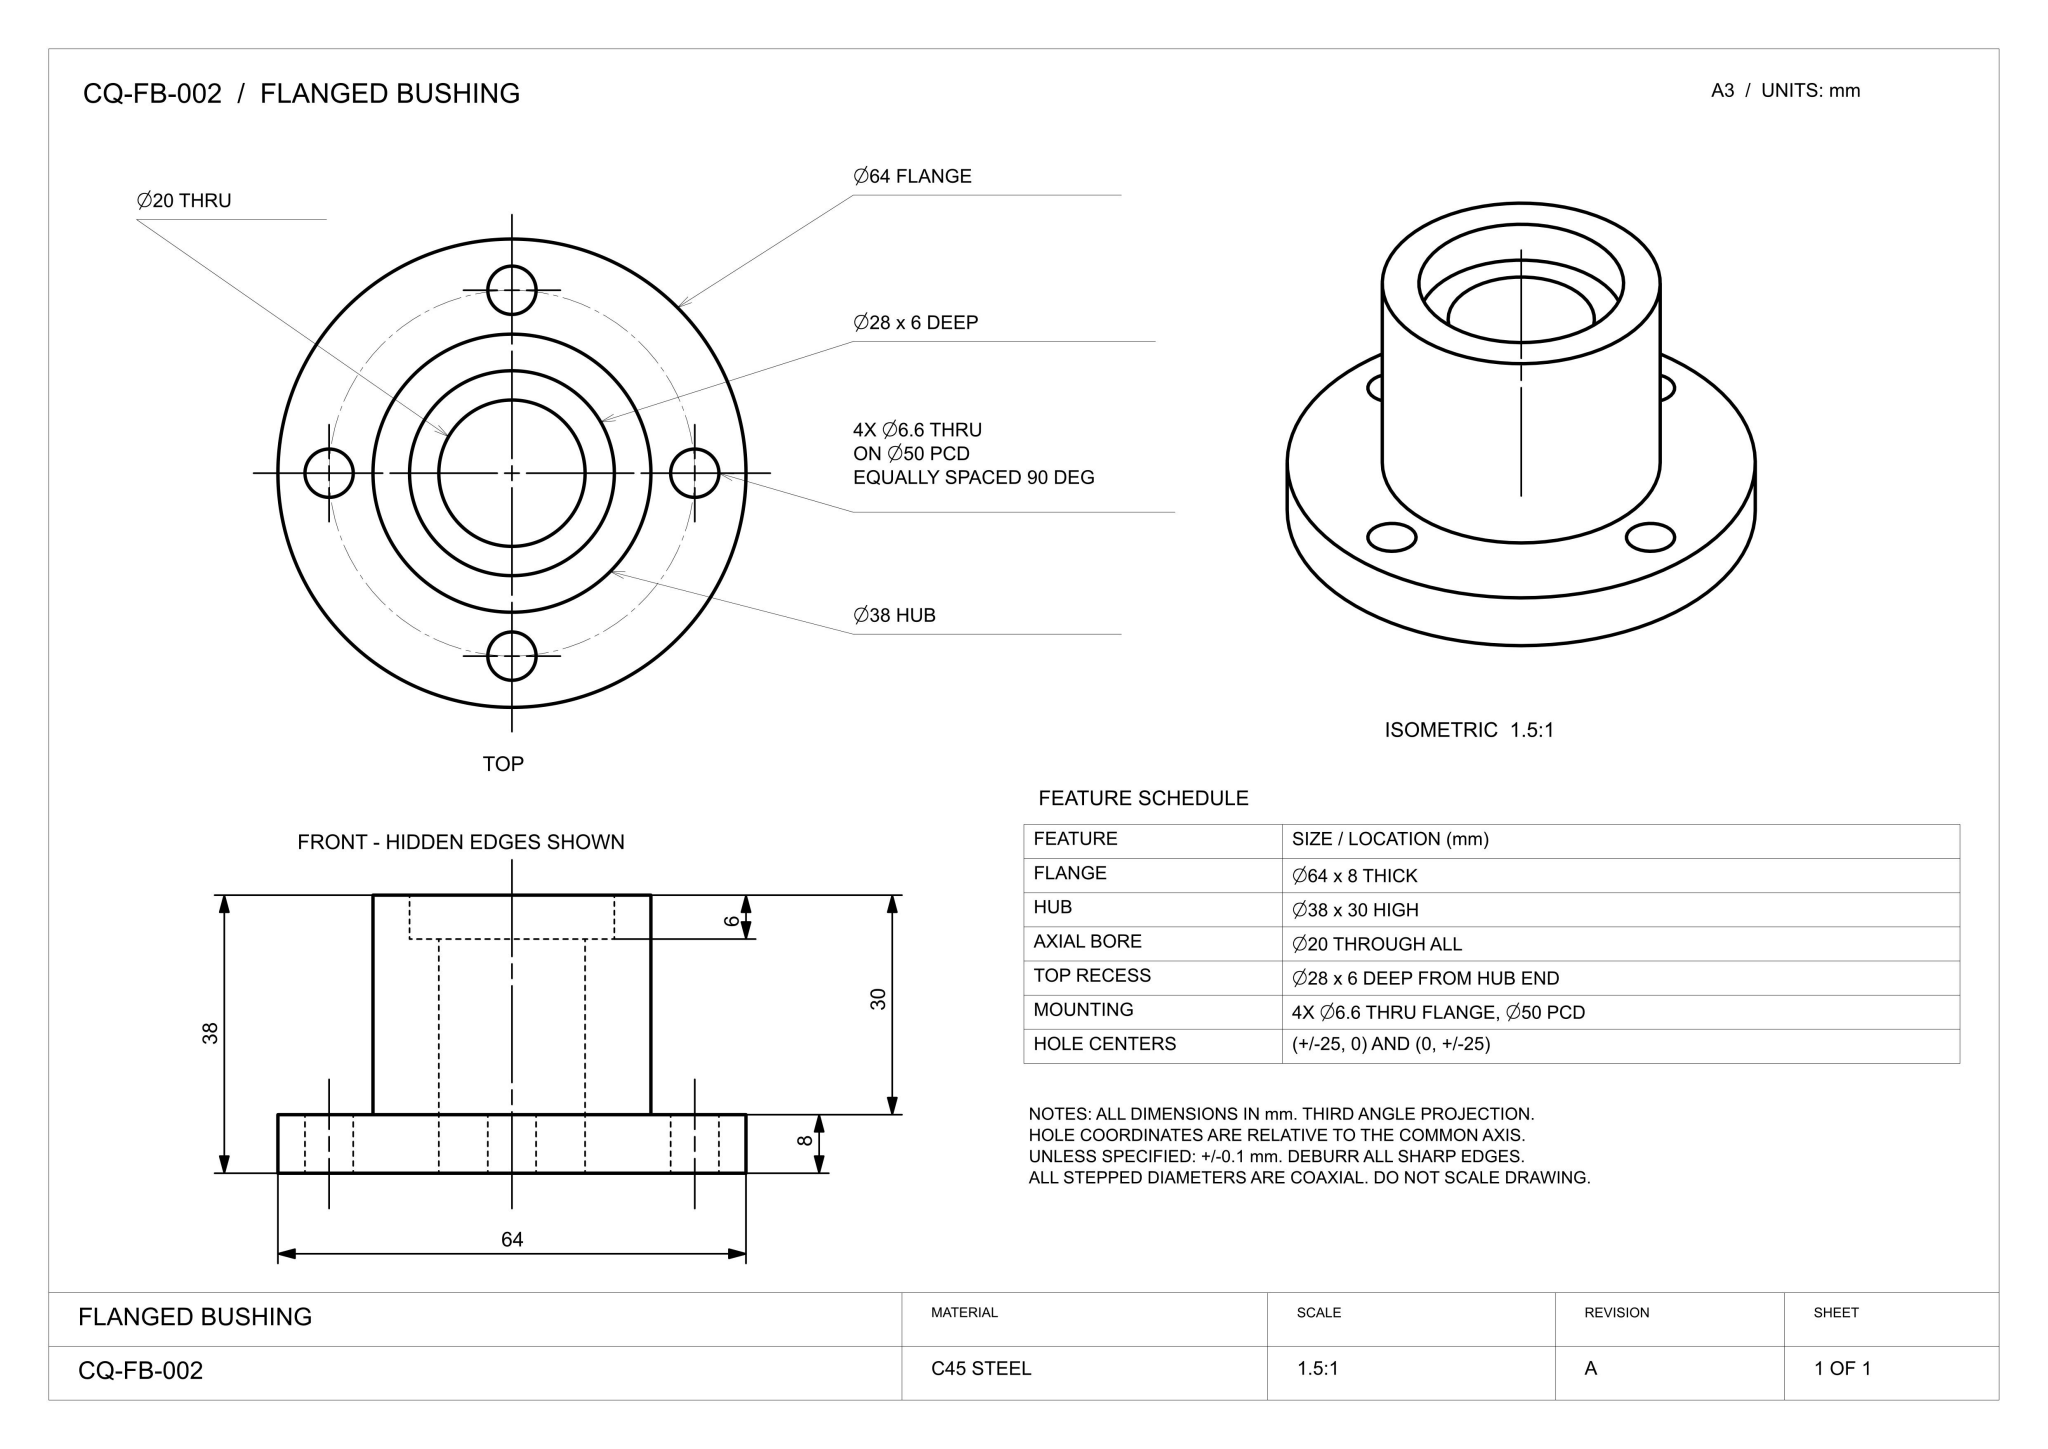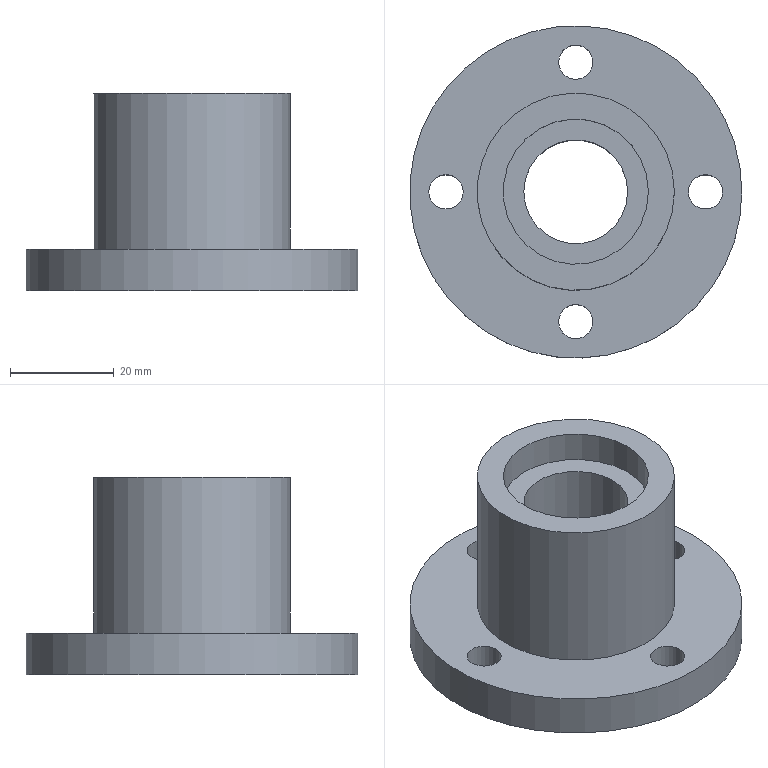Part | NX | mm | 1 solid | 12 faces | box 64 x 64 x 38 mm | volume 44917 mm3 | cylinder 8 | plane 4 | commonest cylinder face diameters 6.6 x4 64 x1 38 x1 20 x1 28 x1
STEP:
#1=CARTESIAN_POINT('',(0.,0.,0.));
#2=DIRECTION('',(0.,0.,1.));
#3=DIRECTION('',(1.,0.,0.));
#4=AXIS2_PLACEMENT_3D('',#1,#2,#3);
#5=(LENGTH_UNIT()NAMED_UNIT(*)SI_UNIT(.MILLI.,.METRE.));
#6=UNCERTAINTY_MEASURE_WITH_UNIT(LENGTH_MEASURE(0.00002),#5,'','');
#7=(NAMED_UNIT(*)PLANE_ANGLE_UNIT()SI_UNIT($,.RADIAN.));
#8=PLANE_ANGLE_MEASURE_WITH_UNIT(PLANE_ANGLE_MEASURE(0.01745),#7);
#9=DIMENSIONAL_EXPONENTS(0.,0.,0.,0.,0.,0.,0.);
#10=(CONVERSION_BASED_UNIT('',#8)NAMED_UNIT(#9)PLANE_ANGLE_UNIT());
#11=(NAMED_UNIT(*)SI_UNIT($,.STERADIAN.)SOLID_ANGLE_UNIT());
#12=(GEOMETRIC_REPRESENTATION_CONTEXT(3)GLOBAL_UNCERTAINTY_ASSIGNED_CONTEXT((#6))GLOBAL_UNIT_ASSIGNED_CONTEXT((#5,#10,#11))REPRESENTATION_CONTEXT('',''));
#13=SHAPE_REPRESENTATION('',(#4),#12);
#14=CARTESIAN_POINT('',(3.3,-25.,8.));
#15=VERTEX_POINT('',#14);
#16=CARTESIAN_POINT('',(0.,-25.,8.));
#17=DIRECTION('',(0.,0.,-1.));
#18=DIRECTION('',(1.,0.,0.));
#19=AXIS2_PLACEMENT_3D('',#16,#17,#18);
#20=CIRCLE('',#19,3.3);
#21=EDGE_CURVE('',#15,#15,#20,.T.);
#22=ORIENTED_EDGE('',*,*,#21,.T.);
#23=EDGE_LOOP('',(#22));
#24=FACE_BOUND('',#23,.T.);
#25=CARTESIAN_POINT('',(-21.7,0.,8.));
#26=VERTEX_POINT('',#25);
#27=CARTESIAN_POINT('',(-25.,0.,8.));
#28=DIRECTION('',(0.,0.,-1.));
#29=DIRECTION('',(1.,0.,0.));
#30=AXIS2_PLACEMENT_3D('',#27,#28,#29);
#31=CIRCLE('',#30,3.3);
#32=EDGE_CURVE('',#26,#26,#31,.T.);
#33=ORIENTED_EDGE('',*,*,#32,.T.);
#34=EDGE_LOOP('',(#33));
#35=FACE_BOUND('',#34,.T.);
#36=CARTESIAN_POINT('',(3.3,25.,8.));
#37=VERTEX_POINT('',#36);
#38=CARTESIAN_POINT('',(0.,25.,8.));
#39=DIRECTION('',(0.,0.,-1.));
#40=DIRECTION('',(1.,0.,0.));
#41=AXIS2_PLACEMENT_3D('',#38,#39,#40);
#42=CIRCLE('',#41,3.3);
#43=EDGE_CURVE('',#37,#37,#42,.T.);
#44=ORIENTED_EDGE('',*,*,#43,.T.);
#45=EDGE_LOOP('',(#44));
#46=FACE_BOUND('',#45,.T.);
#47=CARTESIAN_POINT('',(28.3,0.,8.));
#48=VERTEX_POINT('',#47);
#49=CARTESIAN_POINT('',(25.,0.,8.));
#50=DIRECTION('',(0.,0.,-1.));
#51=DIRECTION('',(1.,0.,0.));
#52=AXIS2_PLACEMENT_3D('',#49,#50,#51);
#53=CIRCLE('',#52,3.3);
#54=EDGE_CURVE('',#48,#48,#53,.T.);
#55=ORIENTED_EDGE('',*,*,#54,.T.);
#56=EDGE_LOOP('',(#55));
#57=FACE_BOUND('',#56,.T.);
#58=CARTESIAN_POINT('',(19.,0.,8.));
#59=VERTEX_POINT('',#58);
#60=CARTESIAN_POINT('',(0.,0.,8.));
#61=DIRECTION('',(0.,0.,1.));
#62=DIRECTION('',(1.,0.,0.));
#63=AXIS2_PLACEMENT_3D('',#60,#61,#62);
#64=CIRCLE('',#63,19.);
#65=EDGE_CURVE('',#59,#59,#64,.T.);
#66=ORIENTED_EDGE('',*,*,#65,.F.);
#67=EDGE_LOOP('',(#66));
#68=FACE_BOUND('',#67,.T.);
#69=CARTESIAN_POINT('',(32.,0.,8.));
#70=VERTEX_POINT('',#69);
#71=CARTESIAN_POINT('',(0.,0.,8.));
#72=DIRECTION('',(0.,0.,-1.));
#73=DIRECTION('',(1.,0.,0.));
#74=AXIS2_PLACEMENT_3D('',#71,#72,#73);
#75=CIRCLE('',#74,32.);
#76=EDGE_CURVE('',#70,#70,#75,.T.);
#77=ORIENTED_EDGE('',*,*,#76,.F.);
#78=EDGE_LOOP('',(#77));
#79=FACE_BOUND('',#78,.T.);
#80=CARTESIAN_POINT('',(0.,0.,8.));
#81=DIRECTION('',(0.,0.,1.));
#82=DIRECTION('',(1.,0.,0.));
#83=AXIS2_PLACEMENT_3D('',#80,#81,#82);
#84=PLANE('',#83);
#85=ADVANCED_FACE('',(#24,#35,#46,#57,#68,#79),#84,.T.);
#86=CARTESIAN_POINT('',(3.3,-25.,0.));
#87=VERTEX_POINT('',#86);
#88=CARTESIAN_POINT('',(0.,-25.,0.));
#89=DIRECTION('',(0.,0.,1.));
#90=DIRECTION('',(1.,0.,0.));
#91=AXIS2_PLACEMENT_3D('',#88,#89,#90);
#92=CIRCLE('',#91,3.3);
#93=EDGE_CURVE('',#87,#87,#92,.T.);
#94=ORIENTED_EDGE('',*,*,#93,.T.);
#95=EDGE_LOOP('',(#94));
#96=FACE_BOUND('',#95,.T.);
#97=CARTESIAN_POINT('',(-21.7,0.,0.));
#98=VERTEX_POINT('',#97);
#99=CARTESIAN_POINT('',(-25.,0.,0.));
#100=DIRECTION('',(0.,0.,1.));
#101=DIRECTION('',(1.,0.,0.));
#102=AXIS2_PLACEMENT_3D('',#99,#100,#101);
#103=CIRCLE('',#102,3.3);
#104=EDGE_CURVE('',#98,#98,#103,.T.);
#105=ORIENTED_EDGE('',*,*,#104,.T.);
#106=EDGE_LOOP('',(#105));
#107=FACE_BOUND('',#106,.T.);
#108=CARTESIAN_POINT('',(3.3,25.,0.));
#109=VERTEX_POINT('',#108);
#110=CARTESIAN_POINT('',(0.,25.,0.));
#111=DIRECTION('',(0.,0.,1.));
#112=DIRECTION('',(1.,0.,0.));
#113=AXIS2_PLACEMENT_3D('',#110,#111,#112);
#114=CIRCLE('',#113,3.3);
#115=EDGE_CURVE('',#109,#109,#114,.T.);
#116=ORIENTED_EDGE('',*,*,#115,.T.);
#117=EDGE_LOOP('',(#116));
#118=FACE_BOUND('',#117,.T.);
#119=CARTESIAN_POINT('',(28.3,0.,0.));
#120=VERTEX_POINT('',#119);
#121=CARTESIAN_POINT('',(25.,0.,0.));
#122=DIRECTION('',(0.,0.,1.));
#123=DIRECTION('',(1.,0.,0.));
#124=AXIS2_PLACEMENT_3D('',#121,#122,#123);
#125=CIRCLE('',#124,3.3);
#126=EDGE_CURVE('',#120,#120,#125,.T.);
#127=ORIENTED_EDGE('',*,*,#126,.T.);
#128=EDGE_LOOP('',(#127));
#129=FACE_BOUND('',#128,.T.);
#130=CARTESIAN_POINT('',(10.,0.,0.));
#131=VERTEX_POINT('',#130);
#132=CARTESIAN_POINT('',(0.,0.,0.));
#133=DIRECTION('',(0.,0.,1.));
#134=DIRECTION('',(1.,0.,0.));
#135=AXIS2_PLACEMENT_3D('',#132,#133,#134);
#136=CIRCLE('',#135,10.);
#137=EDGE_CURVE('',#131,#131,#136,.T.);
#138=ORIENTED_EDGE('',*,*,#137,.T.);
#139=EDGE_LOOP('',(#138));
#140=FACE_BOUND('',#139,.T.);
#141=CARTESIAN_POINT('',(32.,0.,0.));
#142=VERTEX_POINT('',#141);
#143=CARTESIAN_POINT('',(0.,0.,0.));
#144=DIRECTION('',(0.,0.,1.));
#145=DIRECTION('',(1.,0.,0.));
#146=AXIS2_PLACEMENT_3D('',#143,#144,#145);
#147=CIRCLE('',#146,32.);
#148=EDGE_CURVE('',#142,#142,#147,.T.);
#149=ORIENTED_EDGE('',*,*,#148,.F.);
#150=EDGE_LOOP('',(#149));
#151=FACE_BOUND('',#150,.T.);
#152=CARTESIAN_POINT('',(0.,0.,0.));
#153=DIRECTION('',(0.,0.,-1.));
#154=DIRECTION('',(-1.,0.,0.));
#155=AXIS2_PLACEMENT_3D('',#152,#153,#154);
#156=PLANE('',#155);
#157=ADVANCED_FACE('',(#96,#107,#118,#129,#140,#151),#156,.T.);
#158=ORIENTED_EDGE('',*,*,#76,.T.);
#159=EDGE_LOOP('',(#158));
#160=FACE_BOUND('',#159,.T.);
#161=ORIENTED_EDGE('',*,*,#148,.T.);
#162=EDGE_LOOP('',(#161));
#163=FACE_BOUND('',#162,.T.);
#164=CARTESIAN_POINT('',(0.,0.,0.));
#165=DIRECTION('',(0.,0.,1.));
#166=DIRECTION('',(1.,0.,0.));
#167=AXIS2_PLACEMENT_3D('',#164,#165,#166);
#168=CYLINDRICAL_SURFACE('',#167,32.);
#169=ADVANCED_FACE('',(#160,#163),#168,.T.);
#170=CARTESIAN_POINT('',(14.,0.,38.));
#171=VERTEX_POINT('',#170);
#172=CARTESIAN_POINT('',(0.,0.,38.));
#173=DIRECTION('',(0.,0.,-1.));
#174=DIRECTION('',(1.,0.,0.));
#175=AXIS2_PLACEMENT_3D('',#172,#173,#174);
#176=CIRCLE('',#175,14.);
#177=EDGE_CURVE('',#171,#171,#176,.T.);
#178=ORIENTED_EDGE('',*,*,#177,.T.);
#179=EDGE_LOOP('',(#178));
#180=FACE_BOUND('',#179,.T.);
#181=CARTESIAN_POINT('',(19.,0.,38.));
#182=VERTEX_POINT('',#181);
#183=CARTESIAN_POINT('',(0.,0.,38.));
#184=DIRECTION('',(0.,0.,-1.));
#185=DIRECTION('',(1.,0.,0.));
#186=AXIS2_PLACEMENT_3D('',#183,#184,#185);
#187=CIRCLE('',#186,19.);
#188=EDGE_CURVE('',#182,#182,#187,.T.);
#189=ORIENTED_EDGE('',*,*,#188,.F.);
#190=EDGE_LOOP('',(#189));
#191=FACE_BOUND('',#190,.T.);
#192=CARTESIAN_POINT('',(0.,0.,38.));
#193=DIRECTION('',(0.,0.,1.));
#194=DIRECTION('',(1.,0.,0.));
#195=AXIS2_PLACEMENT_3D('',#192,#193,#194);
#196=PLANE('',#195);
#197=ADVANCED_FACE('',(#180,#191),#196,.T.);
#198=ORIENTED_EDGE('',*,*,#188,.T.);
#199=EDGE_LOOP('',(#198));
#200=FACE_BOUND('',#199,.T.);
#201=ORIENTED_EDGE('',*,*,#65,.T.);
#202=EDGE_LOOP('',(#201));
#203=FACE_BOUND('',#202,.T.);
#204=CARTESIAN_POINT('',(0.,0.,8.));
#205=DIRECTION('',(0.,0.,1.));
#206=DIRECTION('',(1.,0.,0.));
#207=AXIS2_PLACEMENT_3D('',#204,#205,#206);
#208=CYLINDRICAL_SURFACE('',#207,19.);
#209=ADVANCED_FACE('',(#200,#203),#208,.T.);
#210=CARTESIAN_POINT('',(-10.,0.,32.));
#211=VERTEX_POINT('',#210);
#212=CARTESIAN_POINT('',(0.,0.,32.));
#213=DIRECTION('',(0.,0.,1.));
#214=DIRECTION('',(-1.,0.,0.));
#215=AXIS2_PLACEMENT_3D('',#212,#213,#214);
#216=CIRCLE('',#215,10.);
#217=EDGE_CURVE('',#211,#211,#216,.T.);
#218=ORIENTED_EDGE('',*,*,#217,.T.);
#219=EDGE_LOOP('',(#218));
#220=FACE_BOUND('',#219,.T.);
#221=ORIENTED_EDGE('',*,*,#137,.F.);
#222=EDGE_LOOP('',(#221));
#223=FACE_BOUND('',#222,.T.);
#224=CARTESIAN_POINT('',(0.,0.,0.));
#225=DIRECTION('',(0.,0.,1.));
#226=DIRECTION('',(1.,0.,0.));
#227=AXIS2_PLACEMENT_3D('',#224,#225,#226);
#228=CYLINDRICAL_SURFACE('',#227,10.);
#229=ADVANCED_FACE('',(#220,#223),#228,.F.);
#230=CARTESIAN_POINT('',(14.,0.,32.));
#231=VERTEX_POINT('',#230);
#232=CARTESIAN_POINT('',(0.,0.,32.));
#233=DIRECTION('',(0.,0.,-1.));
#234=DIRECTION('',(1.,0.,0.));
#235=AXIS2_PLACEMENT_3D('',#232,#233,#234);
#236=CIRCLE('',#235,14.);
#237=EDGE_CURVE('',#231,#231,#236,.T.);
#238=ORIENTED_EDGE('',*,*,#237,.F.);
#239=EDGE_LOOP('',(#238));
#240=FACE_BOUND('',#239,.T.);
#241=ORIENTED_EDGE('',*,*,#217,.F.);
#242=EDGE_LOOP('',(#241));
#243=FACE_BOUND('',#242,.T.);
#244=CARTESIAN_POINT('',(0.,0.,32.));
#245=DIRECTION('',(0.,0.,-1.));
#246=DIRECTION('',(-1.,0.,0.));
#247=AXIS2_PLACEMENT_3D('',#244,#245,#246);
#248=PLANE('',#247);
#249=ADVANCED_FACE('',(#240,#243),#248,.F.);
#250=ORIENTED_EDGE('',*,*,#177,.F.);
#251=EDGE_LOOP('',(#250));
#252=FACE_BOUND('',#251,.T.);
#253=ORIENTED_EDGE('',*,*,#237,.T.);
#254=EDGE_LOOP('',(#253));
#255=FACE_BOUND('',#254,.T.);
#256=CARTESIAN_POINT('',(0.,0.,32.));
#257=DIRECTION('',(0.,0.,1.));
#258=DIRECTION('',(1.,0.,0.));
#259=AXIS2_PLACEMENT_3D('',#256,#257,#258);
#260=CYLINDRICAL_SURFACE('',#259,14.);
#261=ADVANCED_FACE('',(#252,#255),#260,.F.);
#262=ORIENTED_EDGE('',*,*,#54,.F.);
#263=EDGE_LOOP('',(#262));
#264=FACE_BOUND('',#263,.T.);
#265=ORIENTED_EDGE('',*,*,#126,.F.);
#266=EDGE_LOOP('',(#265));
#267=FACE_BOUND('',#266,.T.);
#268=CARTESIAN_POINT('',(25.,0.,0.));
#269=DIRECTION('',(0.,0.,1.));
#270=DIRECTION('',(1.,0.,0.));
#271=AXIS2_PLACEMENT_3D('',#268,#269,#270);
#272=CYLINDRICAL_SURFACE('',#271,3.3);
#273=ADVANCED_FACE('',(#264,#267),#272,.F.);
#274=ORIENTED_EDGE('',*,*,#43,.F.);
#275=EDGE_LOOP('',(#274));
#276=FACE_BOUND('',#275,.T.);
#277=ORIENTED_EDGE('',*,*,#115,.F.);
#278=EDGE_LOOP('',(#277));
#279=FACE_BOUND('',#278,.T.);
#280=CARTESIAN_POINT('',(0.,25.,0.));
#281=DIRECTION('',(0.,0.,1.));
#282=DIRECTION('',(1.,0.,0.));
#283=AXIS2_PLACEMENT_3D('',#280,#281,#282);
#284=CYLINDRICAL_SURFACE('',#283,3.3);
#285=ADVANCED_FACE('',(#276,#279),#284,.F.);
#286=ORIENTED_EDGE('',*,*,#32,.F.);
#287=EDGE_LOOP('',(#286));
#288=FACE_BOUND('',#287,.T.);
#289=ORIENTED_EDGE('',*,*,#104,.F.);
#290=EDGE_LOOP('',(#289));
#291=FACE_BOUND('',#290,.T.);
#292=CARTESIAN_POINT('',(-25.,0.,0.));
#293=DIRECTION('',(0.,0.,1.));
#294=DIRECTION('',(1.,0.,0.));
#295=AXIS2_PLACEMENT_3D('',#292,#293,#294);
#296=CYLINDRICAL_SURFACE('',#295,3.3);
#297=ADVANCED_FACE('',(#288,#291),#296,.F.);
#298=ORIENTED_EDGE('',*,*,#21,.F.);
#299=EDGE_LOOP('',(#298));
#300=FACE_BOUND('',#299,.T.);
#301=ORIENTED_EDGE('',*,*,#93,.F.);
#302=EDGE_LOOP('',(#301));
#303=FACE_BOUND('',#302,.T.);
#304=CARTESIAN_POINT('',(0.,-25.,0.));
#305=DIRECTION('',(0.,0.,1.));
#306=DIRECTION('',(1.,0.,0.));
#307=AXIS2_PLACEMENT_3D('',#304,#305,#306);
#308=CYLINDRICAL_SURFACE('',#307,3.3);
#309=ADVANCED_FACE('',(#300,#303),#308,.F.);
#310=CLOSED_SHELL('',(#85,#157,#169,#197,#209,#229,#249,#261,#273,#285,#297,#309));
#311=MANIFOLD_SOLID_BREP('',#310);
#312=ADVANCED_BREP_SHAPE_REPRESENTATION('',(#311),#12);
#313=SHAPE_REPRESENTATION_RELATIONSHIP('','',#13,#312);
#314=PRESENTATION_LAYER_ASSIGNMENT('','',(#311));
#315=COLOUR_RGB('',0.6118,0.6588,0.6706);
#316=FILL_AREA_STYLE_COLOUR('',#315);
#317=FILL_AREA_STYLE('',(#316));
#318=SURFACE_STYLE_FILL_AREA(#317);
#319=SURFACE_SIDE_STYLE('',(#318));
#320=SURFACE_STYLE_USAGE(.BOTH.,#319);
#321=PRESENTATION_STYLE_ASSIGNMENT((#320));
#322=STYLED_ITEM('',(#321),#311);
#323=MECHANICAL_DESIGN_GEOMETRIC_PRESENTATION_REPRESENTATION('',(#322),#12);